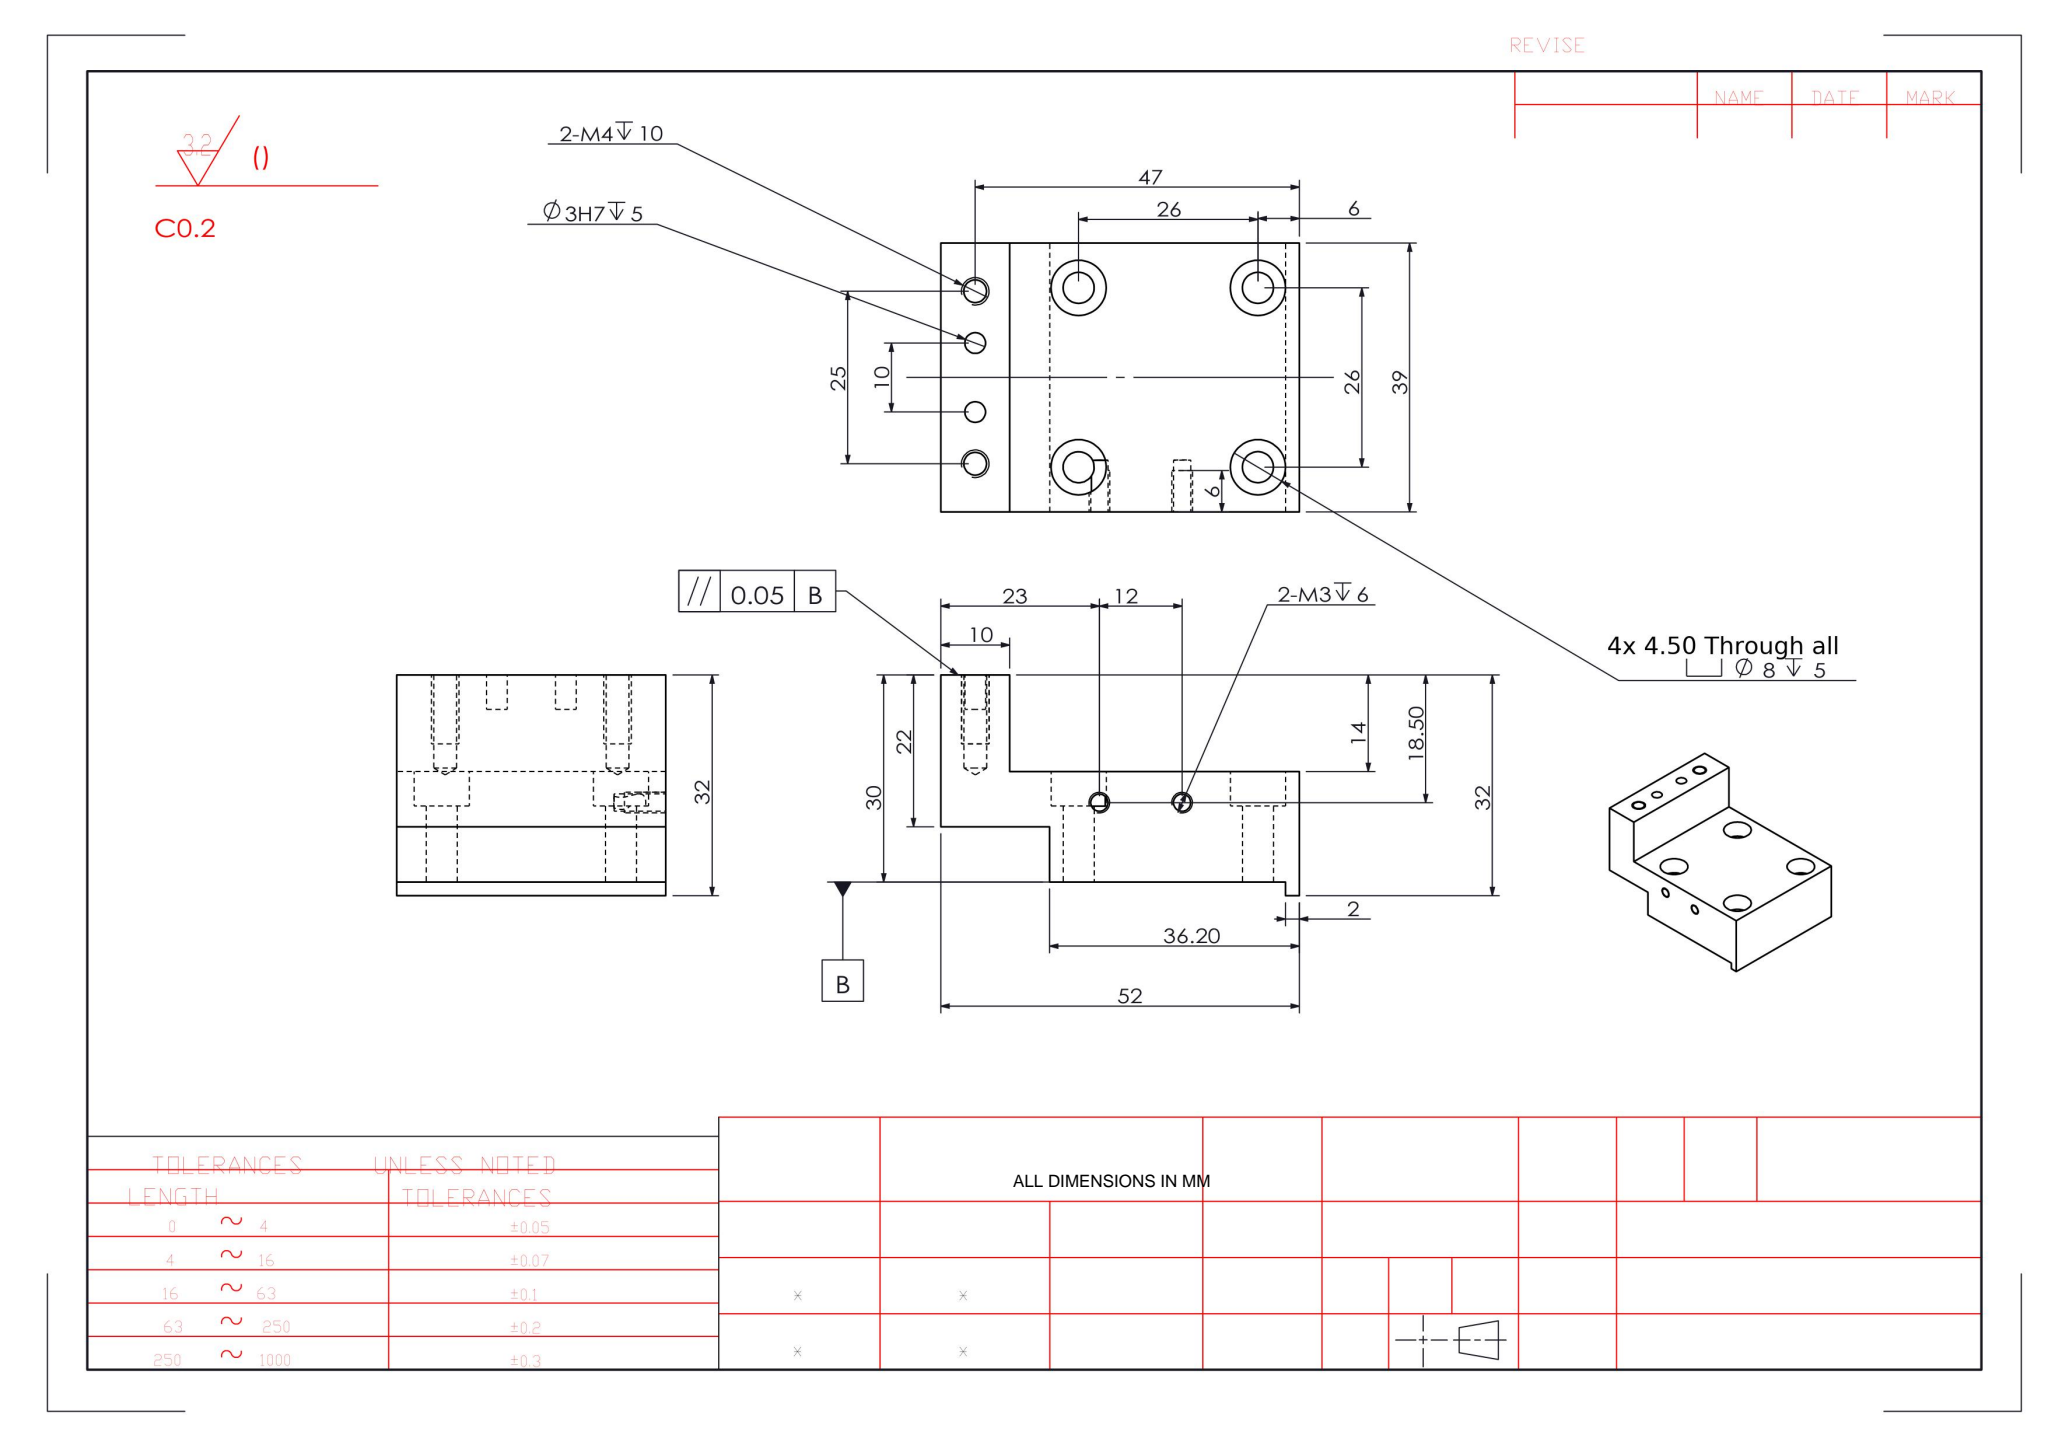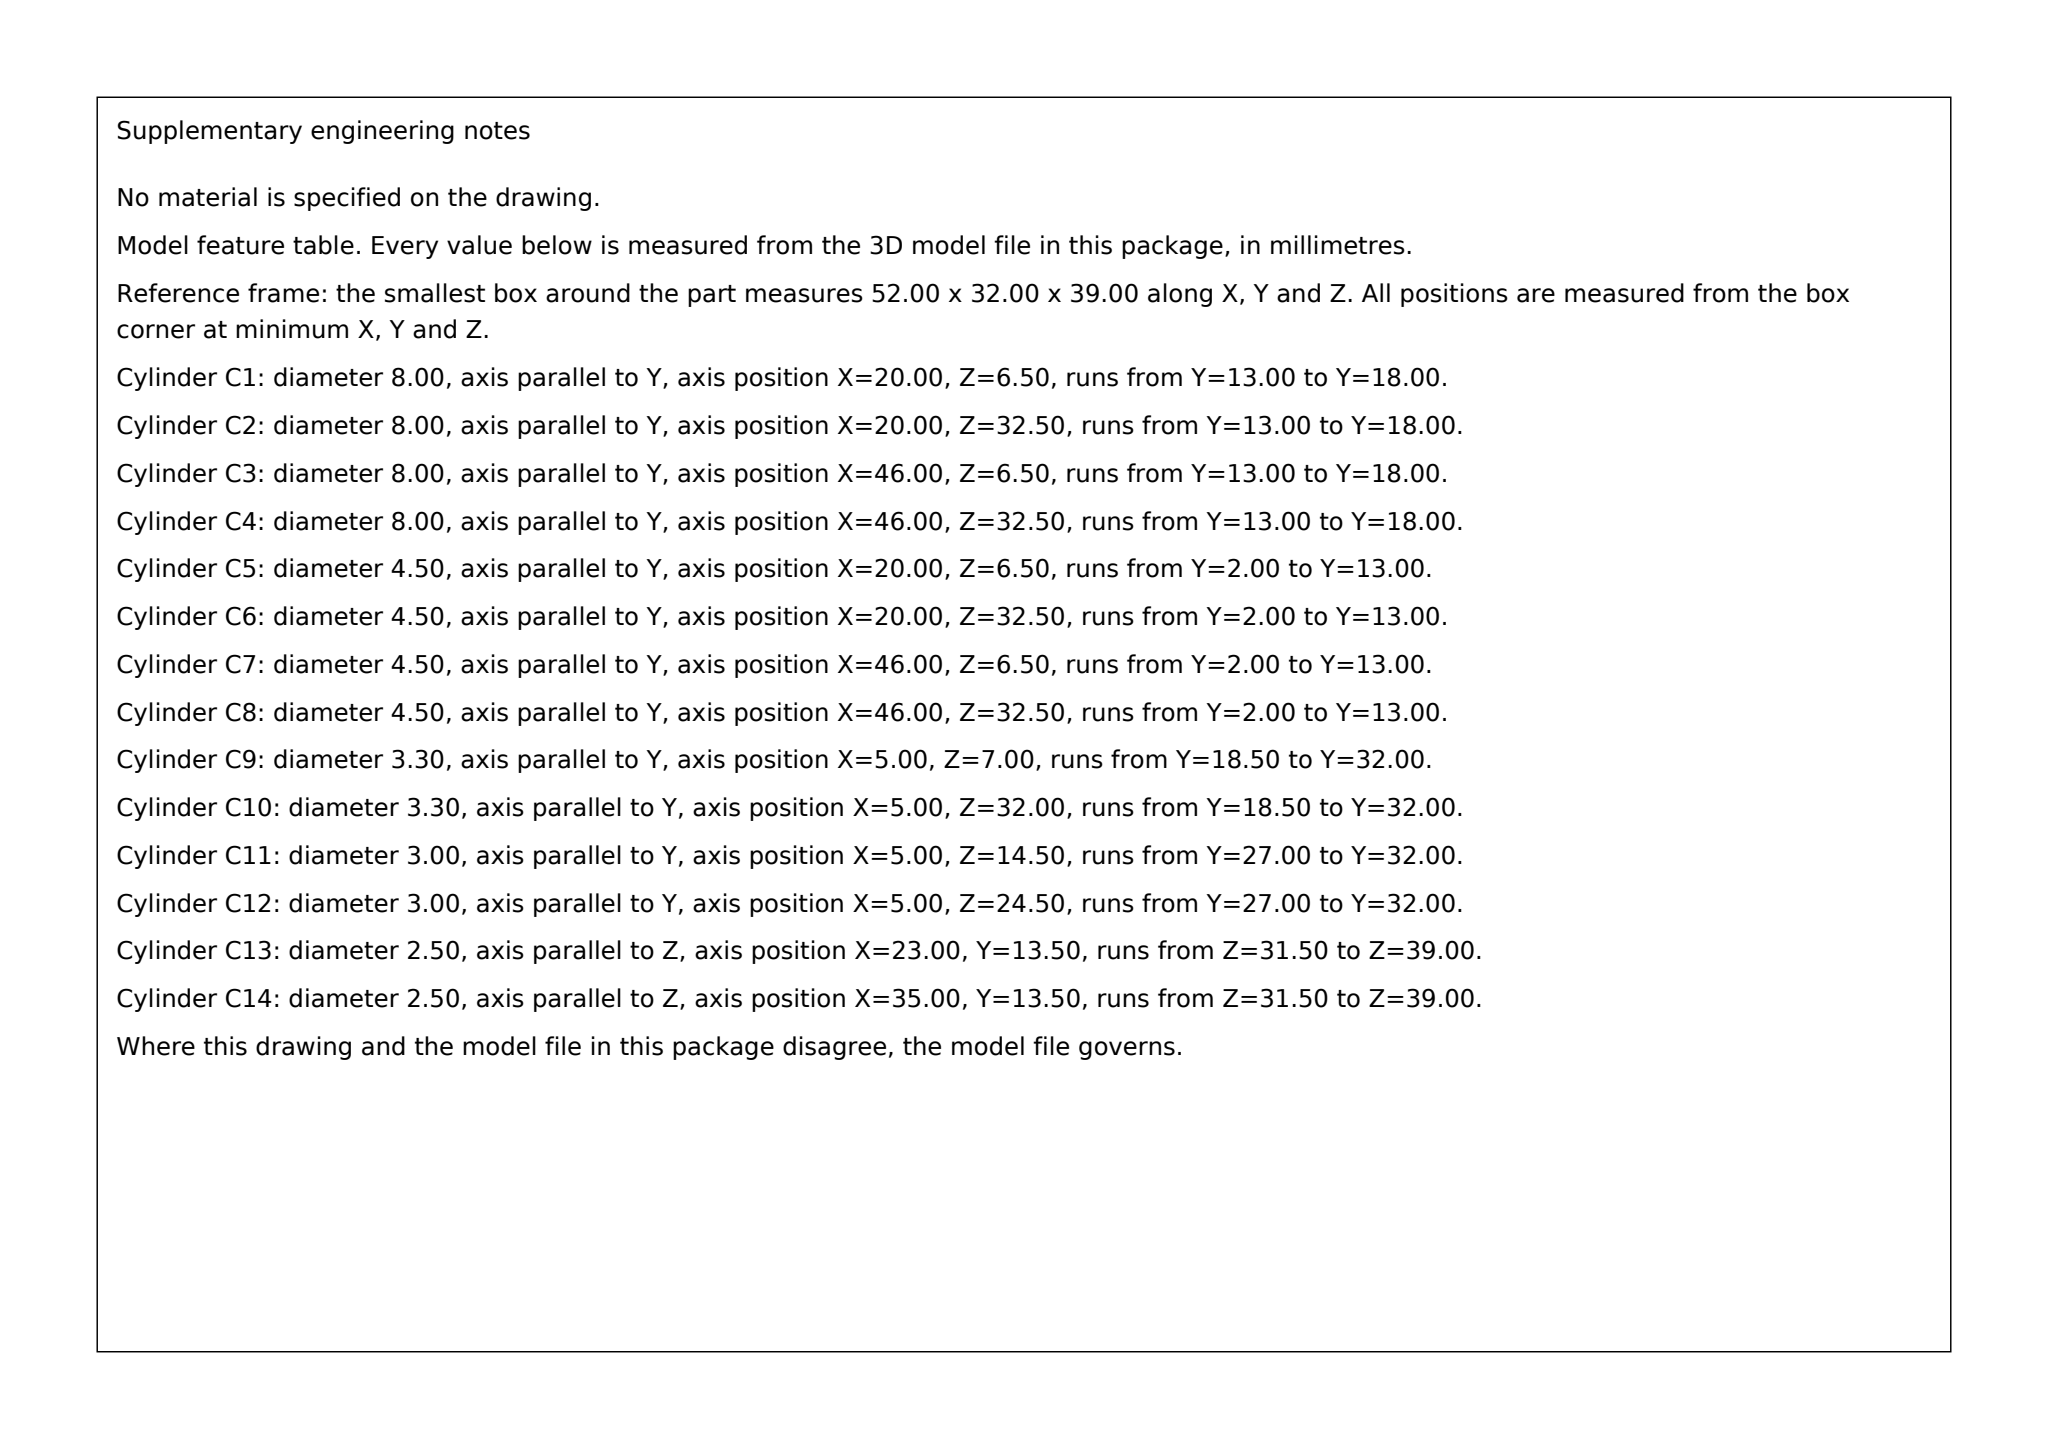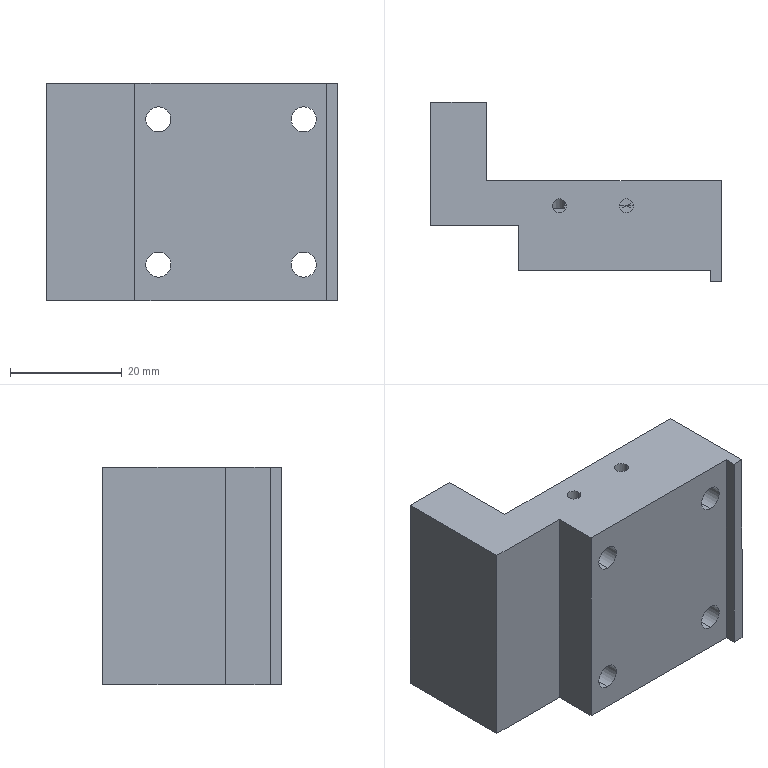Part | SolidWorks | mm | 1 solid | 54 faces | box 52 x 32 x 39 mm | volume 31061 mm3 | cylinder 28 | plane 18 | cone 8 | commonest cylinder face diameters 8 x8 4.5 x8 2.5 x4 3 x4 3.3 x4
build123d program:
from build123d import *

# Parameters (mm, degrees)
BOSS_EXTRUDE1_DEPTH                             = 39
M4_HEX_SOCKET_HEAD_CAP_SCREW_CBORE1_D           = 4.5
M4_HEX_SOCKET_HEAD_CAP_SCREW_CBORE1_CBORE_D     = 8
M4_HEX_SOCKET_HEAD_CAP_SCREW_CBORE1_CBORE_DEPTH = 5
M4_TAPPED_HOLE2_D                               = 3.3
M4_TAPPED_HOLE2_DEPTH                           = 13.5
M4_TAPPED_HOLE2_TIP                             = 0.9914
SKETCH8_R                                       = 1.5
CUT_EXTRUDE1_DEPTH                              = 5
SKETCH11_W                                      = 147.804
SKETCH11_H                                      = 73.676
CUT_EXTRUDE2_DEPTH                              = 104.175
M3_TAPPED_HOLE2_D                               = 2.5
M3_TAPPED_HOLE2_DEPTH                           = 7.5
M3_TAPPED_HOLE2_TIP                             = 0.05458


with BuildPart() as part:
    # Sketch1 → Boss-Extrude1 (new body)
    with BuildSketch(Plane.XY):
        Polygon((80, 32), (90, 32), (90, 10), (74.2, 10), (74.2, 2), (40, 2), (40, 0), (-40, 0), (-40, 2), (-74.2, 2), (-74.2, 10), (-90, 10), (-90, 32), (-80, 32), (-80, 18), (80, 18), align=None)
    extrude(amount=BOSS_EXTRUDE1_DEPTH)

    # M4 Hex Socket Head Cap Screw CBORE1 (through all)
    with Locations(Plane(origin=(-70, 18, 32.5), x_dir=(1, 0, 0), z_dir=(0, 1, 0))):
        with Locations((0, 0), (26, 0), (26, 26), (0, 26), (114, 0), (140, 0), (114, 26), (140, 26)):
            CounterBoreHole(M4_HEX_SOCKET_HEAD_CAP_SCREW_CBORE1_D / 2, M4_HEX_SOCKET_HEAD_CAP_SCREW_CBORE1_CBORE_D / 2, M4_HEX_SOCKET_HEAD_CAP_SCREW_CBORE1_CBORE_DEPTH)

    # M4 Tapped Hole2
    with Locations(Plane(origin=(85, 32, 7), x_dir=(0, 0, 1), z_dir=(0, 1, 0))):
        with Locations((0, 0), (25, 0), (0, -170), (25, -170)):
            Hole(M4_TAPPED_HOLE2_D / 2, depth=M4_TAPPED_HOLE2_DEPTH)
            with Locations((0, 0, -(M4_TAPPED_HOLE2_DEPTH + M4_TAPPED_HOLE2_TIP / 2))):  # 118° drill point
                Cone(0, M4_TAPPED_HOLE2_D / 2, M4_TAPPED_HOLE2_TIP, mode=Mode.SUBTRACT)

    # Sketch8 → Cut-Extrude1 (cut)
    with BuildSketch(Plane(origin=(0, 32, 0), x_dir=(1, 0, 0), z_dir=(0, 1, 0))):
        with Locations(Location((85, -14.5, 0), (0, 0, 270))):
            Circle(SKETCH8_R)
        with Locations(Location((85, -24.5, 0), (0, 0, 270))):
            Circle(SKETCH8_R)
        with Locations(Location((-85, -14.5, 0), (0, 0, 270))):
            Circle(SKETCH8_R)
        with Locations(Location((-85, -24.5, 0), (0, 0, 270))):
            Circle(SKETCH8_R)
    extrude(amount=-CUT_EXTRUDE1_DEPTH, mode=Mode.SUBTRACT)

    # Sketch11 → Cut-Extrude2 (cut, through all)
    with BuildSketch(Plane.XY.offset(39)):
        with Locations((35.902, 15.171)):
            Rectangle(SKETCH11_W, SKETCH11_H)
    extrude(amount=-CUT_EXTRUDE2_DEPTH, mode=Mode.SUBTRACT)

    # M3 Tapped Hole2
    with Locations(Plane.XY.offset(39)):
        with Locations((-67, 13.5), (-55, 13.5)):
            Hole(M3_TAPPED_HOLE2_D / 2, depth=M3_TAPPED_HOLE2_DEPTH)
            with Locations((0, 0, -(M3_TAPPED_HOLE2_DEPTH + M3_TAPPED_HOLE2_TIP / 2))):  # 175° drill point
                Cone(0, M3_TAPPED_HOLE2_D / 2, M3_TAPPED_HOLE2_TIP, mode=Mode.SUBTRACT)


solid = part.part